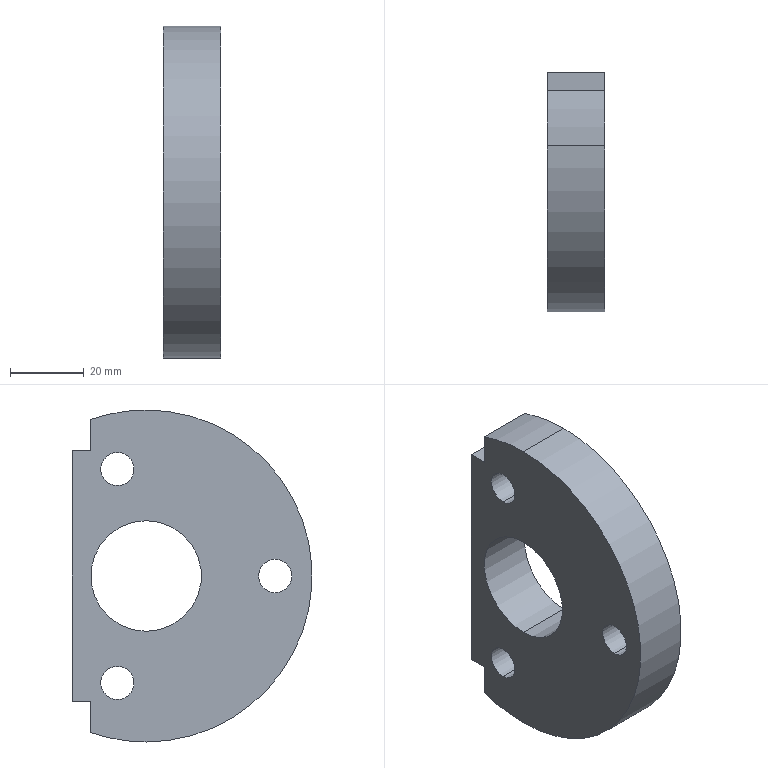Component | SolidWorks | 2SemicircularSupportPlate-1 | 1 solid | 27 faces | box 15.5 x 65 x 90 mm | volume 59022 mm3 | cylinder 17 | plane 10 | commonest cylinder face diameters 14 x6 9 x6 90 x3 30 x2
build123d program:
from build123d import *

# Parameters (mm, degrees)
BOSS_EXTRUDE1_DEPTH     = 15.5
CUT_EXTRUDE1_DEPTH      = 66.5
CUT_EXTRUDE1_DEPTH_BACK = 66.5
SKETCH2_R               = 15
HOLE1_D                 = 9
HOLE1_DEPTH             = 100
HOLE1_CBORE_D           = 14
HOLE1_CBORE_DEPTH       = 8


with BuildPart() as part:
    # Sketch1 → Boss-Extrude1 (new body)
    with BuildSketch(Plane.XY):
        with BuildLine():
            Line((-42.426, 15), (-34, 15))
            Line((-34, 15), (-34, 20))
            Line((-34, 20), (34, 20))
            Line((34, 20), (34, 15))
            Line((34, 15), (42.426, 15))
            ThreePointArc((42.426, 15), (0, -45), (-42.426, 15))
        make_face()
    extrude(amount=BOSS_EXTRUDE1_DEPTH)

    # Sketch2 → Cut-Extrude1 (cut, two sides: drawn at the far end of the back side and taken through both)
    with BuildSketch(Plane.XY.offset(15.5).offset(-CUT_EXTRUDE1_DEPTH_BACK)):
        Circle(SKETCH2_R)
    extrude(amount=CUT_EXTRUDE1_DEPTH + CUT_EXTRUDE1_DEPTH_BACK, mode=Mode.SUBTRACT)

    # Hole1
    with Locations(Plane.XY.offset(15.5)):
        with Locations((-28.978, 7.765), (28.978, 7.765), (0, -35)):
            CounterBoreHole(HOLE1_D / 2, HOLE1_CBORE_D / 2, HOLE1_CBORE_DEPTH, depth=HOLE1_DEPTH)


solid = part.part

# Placed as in the assembly
solid = solid.moved(Location((200, 65, 0), (0, 90, 0)))
STEP:
#1=COLOUR_RGB('',0.7922,0.8196,0.9333);
#2=FILL_AREA_STYLE_COLOUR('',#1);
#3=FILL_AREA_STYLE('',(#2));
#4=SURFACE_STYLE_FILL_AREA(#3);
#5=SURFACE_SIDE_STYLE('',(#4));
#6=SURFACE_STYLE_USAGE(.BOTH.,#5);
#7=PRESENTATION_STYLE_ASSIGNMENT((#6));
#8=CARTESIAN_POINT('',(8.169,1.181,0.2756));
#9=VERTEX_POINT('',#8);
#10=CARTESIAN_POINT('',(8.169,1.181,-0.2756));
#11=VERTEX_POINT('',#10);
#12=CARTESIAN_POINT('',(8.169,1.181,0.));
#13=DIRECTION('',(1.,-0.,-0.));
#14=DIRECTION('',(0.,-0.,-1.));
#15=AXIS2_PLACEMENT_3D('',#12,#13,#14);
#16=CIRCLE('',#15,0.2756);
#17=EDGE_CURVE('',#9,#11,#16,.T.);
#18=ORIENTED_EDGE('',*,*,#17,.F.);
#19=CARTESIAN_POINT('',(8.484,1.181,0.2756));
#20=VERTEX_POINT('',#19);
#21=CARTESIAN_POINT('',(8.484,1.181,0.2756));
#22=DIRECTION('',(1.,-0.,-0.));
#23=VECTOR('',#22,39.37);
#24=LINE('',#21,#23);
#25=EDGE_CURVE('',#9,#20,#24,.T.);
#26=ORIENTED_EDGE('',*,*,#25,.T.);
#27=CARTESIAN_POINT('',(8.484,1.181,-0.2756));
#28=VERTEX_POINT('',#27);
#29=CARTESIAN_POINT('',(8.484,1.181,0.));
#30=DIRECTION('',(1.,-0.,-0.));
#31=DIRECTION('',(0.,-0.,-1.));
#32=AXIS2_PLACEMENT_3D('',#29,#30,#31);
#33=CIRCLE('',#32,0.2756);
#34=EDGE_CURVE('',#20,#28,#33,.T.);
#35=ORIENTED_EDGE('',*,*,#34,.T.);
#36=CARTESIAN_POINT('',(8.484,1.181,-0.2756));
#37=DIRECTION('',(1.,-0.,-0.));
#38=VECTOR('',#37,39.37);
#39=LINE('',#36,#38);
#40=EDGE_CURVE('',#11,#28,#39,.T.);
#41=ORIENTED_EDGE('',*,*,#40,.F.);
#42=EDGE_LOOP('',(#18,#26,#35,#41));
#43=FACE_OUTER_BOUND('',#42,.T.);
#44=CARTESIAN_POINT('',(8.484,1.181,0.));
#45=DIRECTION('',(1.,-0.,-0.));
#46=DIRECTION('',(0.,-0.,-1.));
#47=AXIS2_PLACEMENT_3D('',#44,#45,#46);
#48=CYLINDRICAL_SURFACE('',#47,0.2756);
#49=ADVANCED_FACE('',(#43),#48,.F.);
#50=CARTESIAN_POINT('',(7.874,1.181,0.1772));
#51=VERTEX_POINT('',#50);
#52=CARTESIAN_POINT('',(7.874,1.181,-0.1772));
#53=VERTEX_POINT('',#52);
#54=CARTESIAN_POINT('',(7.874,1.181,0.));
#55=DIRECTION('',(1.,-0.,-0.));
#56=DIRECTION('',(0.,-0.,-1.));
#57=AXIS2_PLACEMENT_3D('',#54,#55,#56);
#58=CIRCLE('',#57,0.1772);
#59=EDGE_CURVE('',#51,#53,#58,.T.);
#60=ORIENTED_EDGE('',*,*,#59,.F.);
#61=CARTESIAN_POINT('',(8.169,1.181,0.1772));
#62=VERTEX_POINT('',#61);
#63=CARTESIAN_POINT('',(8.484,1.181,0.1772));
#64=DIRECTION('',(1.,-0.,-0.));
#65=VECTOR('',#64,39.37);
#66=LINE('',#63,#65);
#67=EDGE_CURVE('',#51,#62,#66,.T.);
#68=ORIENTED_EDGE('',*,*,#67,.T.);
#69=CARTESIAN_POINT('',(8.169,1.181,-0.1772));
#70=VERTEX_POINT('',#69);
#71=CARTESIAN_POINT('',(8.169,1.181,0.));
#72=DIRECTION('',(1.,-0.,-0.));
#73=DIRECTION('',(0.,-0.,-1.));
#74=AXIS2_PLACEMENT_3D('',#71,#72,#73);
#75=CIRCLE('',#74,0.1772);
#76=EDGE_CURVE('',#62,#70,#75,.T.);
#77=ORIENTED_EDGE('',*,*,#76,.T.);
#78=CARTESIAN_POINT('',(8.484,1.181,-0.1772));
#79=DIRECTION('',(1.,-0.,-0.));
#80=VECTOR('',#79,39.37);
#81=LINE('',#78,#80);
#82=EDGE_CURVE('',#53,#70,#81,.T.);
#83=ORIENTED_EDGE('',*,*,#82,.F.);
#84=EDGE_LOOP('',(#60,#68,#77,#83));
#85=FACE_OUTER_BOUND('',#84,.T.);
#86=CARTESIAN_POINT('',(8.484,1.181,0.));
#87=DIRECTION('',(1.,-0.,-0.));
#88=DIRECTION('',(0.,-0.,-1.));
#89=AXIS2_PLACEMENT_3D('',#86,#87,#88);
#90=CYLINDRICAL_SURFACE('',#89,0.1772);
#91=ADVANCED_FACE('',(#85),#90,.F.);
#92=CARTESIAN_POINT('',(8.169,2.865,-0.8653));
#93=VERTEX_POINT('',#92);
#94=CARTESIAN_POINT('',(8.169,2.865,-1.416));
#95=VERTEX_POINT('',#94);
#96=CARTESIAN_POINT('',(8.169,2.865,-1.141));
#97=DIRECTION('',(1.,-0.,-0.));
#98=DIRECTION('',(0.,-0.,-1.));
#99=AXIS2_PLACEMENT_3D('',#96,#97,#98);
#100=CIRCLE('',#99,0.2756);
#101=EDGE_CURVE('',#93,#95,#100,.T.);
#102=ORIENTED_EDGE('',*,*,#101,.F.);
#103=CARTESIAN_POINT('',(8.484,2.865,-0.8653));
#104=VERTEX_POINT('',#103);
#105=CARTESIAN_POINT('',(8.484,2.865,-0.8653));
#106=DIRECTION('',(1.,-0.,-0.));
#107=VECTOR('',#106,39.37);
#108=LINE('',#105,#107);
#109=EDGE_CURVE('',#93,#104,#108,.T.);
#110=ORIENTED_EDGE('',*,*,#109,.T.);
#111=CARTESIAN_POINT('',(8.484,2.865,-1.416));
#112=VERTEX_POINT('',#111);
#113=CARTESIAN_POINT('',(8.484,2.865,-1.141));
#114=DIRECTION('',(1.,-0.,-0.));
#115=DIRECTION('',(0.,-0.,-1.));
#116=AXIS2_PLACEMENT_3D('',#113,#114,#115);
#117=CIRCLE('',#116,0.2756);
#118=EDGE_CURVE('',#104,#112,#117,.T.);
#119=ORIENTED_EDGE('',*,*,#118,.T.);
#120=CARTESIAN_POINT('',(8.484,2.865,-1.416));
#121=DIRECTION('',(1.,-0.,-0.));
#122=VECTOR('',#121,39.37);
#123=LINE('',#120,#122);
#124=EDGE_CURVE('',#95,#112,#123,.T.);
#125=ORIENTED_EDGE('',*,*,#124,.F.);
#126=EDGE_LOOP('',(#102,#110,#119,#125));
#127=FACE_OUTER_BOUND('',#126,.T.);
#128=CARTESIAN_POINT('',(8.484,2.865,-1.141));
#129=DIRECTION('',(1.,-0.,-0.));
#130=DIRECTION('',(0.,-0.,-1.));
#131=AXIS2_PLACEMENT_3D('',#128,#129,#130);
#132=CYLINDRICAL_SURFACE('',#131,0.2756);
#133=ADVANCED_FACE('',(#127),#132,.F.);
#134=CARTESIAN_POINT('',(7.874,2.865,-0.9637));
#135=VERTEX_POINT('',#134);
#136=CARTESIAN_POINT('',(7.874,2.865,-1.318));
#137=VERTEX_POINT('',#136);
#138=CARTESIAN_POINT('',(7.874,2.865,-1.141));
#139=DIRECTION('',(1.,-0.,-0.));
#140=DIRECTION('',(0.,-0.,-1.));
#141=AXIS2_PLACEMENT_3D('',#138,#139,#140);
#142=CIRCLE('',#141,0.1772);
#143=EDGE_CURVE('',#135,#137,#142,.T.);
#144=ORIENTED_EDGE('',*,*,#143,.F.);
#145=CARTESIAN_POINT('',(8.169,2.865,-0.9637));
#146=VERTEX_POINT('',#145);
#147=CARTESIAN_POINT('',(8.484,2.865,-0.9637));
#148=DIRECTION('',(1.,-0.,-0.));
#149=VECTOR('',#148,39.37);
#150=LINE('',#147,#149);
#151=EDGE_CURVE('',#135,#146,#150,.T.);
#152=ORIENTED_EDGE('',*,*,#151,.T.);
#153=CARTESIAN_POINT('',(8.169,2.865,-1.318));
#154=VERTEX_POINT('',#153);
#155=CARTESIAN_POINT('',(8.169,2.865,-1.141));
#156=DIRECTION('',(1.,-0.,-0.));
#157=DIRECTION('',(0.,-0.,-1.));
#158=AXIS2_PLACEMENT_3D('',#155,#156,#157);
#159=CIRCLE('',#158,0.1772);
#160=EDGE_CURVE('',#146,#154,#159,.T.);
#161=ORIENTED_EDGE('',*,*,#160,.T.);
#162=CARTESIAN_POINT('',(8.484,2.865,-1.318));
#163=DIRECTION('',(1.,-0.,-0.));
#164=VECTOR('',#163,39.37);
#165=LINE('',#162,#164);
#166=EDGE_CURVE('',#137,#154,#165,.T.);
#167=ORIENTED_EDGE('',*,*,#166,.F.);
#168=EDGE_LOOP('',(#144,#152,#161,#167));
#169=FACE_OUTER_BOUND('',#168,.T.);
#170=CARTESIAN_POINT('',(8.484,2.865,-1.141));
#171=DIRECTION('',(1.,-0.,-0.));
#172=DIRECTION('',(0.,-0.,-1.));
#173=AXIS2_PLACEMENT_3D('',#170,#171,#172);
#174=CYLINDRICAL_SURFACE('',#173,0.1772);
#175=ADVANCED_FACE('',(#169),#174,.F.);
#176=CARTESIAN_POINT('',(8.169,2.865,1.416));
#177=VERTEX_POINT('',#176);
#178=CARTESIAN_POINT('',(8.169,2.865,0.8653));
#179=VERTEX_POINT('',#178);
#180=CARTESIAN_POINT('',(8.169,2.865,1.141));
#181=DIRECTION('',(1.,-0.,-0.));
#182=DIRECTION('',(0.,-0.,-1.));
#183=AXIS2_PLACEMENT_3D('',#180,#181,#182);
#184=CIRCLE('',#183,0.2756);
#185=EDGE_CURVE('',#177,#179,#184,.T.);
#186=ORIENTED_EDGE('',*,*,#185,.F.);
#187=CARTESIAN_POINT('',(8.484,2.865,1.416));
#188=VERTEX_POINT('',#187);
#189=CARTESIAN_POINT('',(8.484,2.865,1.416));
#190=DIRECTION('',(1.,-0.,-0.));
#191=VECTOR('',#190,39.37);
#192=LINE('',#189,#191);
#193=EDGE_CURVE('',#177,#188,#192,.T.);
#194=ORIENTED_EDGE('',*,*,#193,.T.);
#195=CARTESIAN_POINT('',(8.484,2.865,0.8653));
#196=VERTEX_POINT('',#195);
#197=CARTESIAN_POINT('',(8.484,2.865,1.141));
#198=DIRECTION('',(1.,-0.,-0.));
#199=DIRECTION('',(0.,-0.,-1.));
#200=AXIS2_PLACEMENT_3D('',#197,#198,#199);
#201=CIRCLE('',#200,0.2756);
#202=EDGE_CURVE('',#188,#196,#201,.T.);
#203=ORIENTED_EDGE('',*,*,#202,.T.);
#204=CARTESIAN_POINT('',(8.484,2.865,0.8653));
#205=DIRECTION('',(1.,-0.,-0.));
#206=VECTOR('',#205,39.37);
#207=LINE('',#204,#206);
#208=EDGE_CURVE('',#179,#196,#207,.T.);
#209=ORIENTED_EDGE('',*,*,#208,.F.);
#210=EDGE_LOOP('',(#186,#194,#203,#209));
#211=FACE_OUTER_BOUND('',#210,.T.);
#212=CARTESIAN_POINT('',(8.484,2.865,1.141));
#213=DIRECTION('',(1.,-0.,-0.));
#214=DIRECTION('',(0.,-0.,-1.));
#215=AXIS2_PLACEMENT_3D('',#212,#213,#214);
#216=CYLINDRICAL_SURFACE('',#215,0.2756);
#217=ADVANCED_FACE('',(#211),#216,.F.);
#218=CARTESIAN_POINT('',(7.874,2.865,1.318));
#219=VERTEX_POINT('',#218);
#220=CARTESIAN_POINT('',(7.874,2.865,0.9637));
#221=VERTEX_POINT('',#220);
#222=CARTESIAN_POINT('',(7.874,2.865,1.141));
#223=DIRECTION('',(1.,-0.,-0.));
#224=DIRECTION('',(0.,-0.,-1.));
#225=AXIS2_PLACEMENT_3D('',#222,#223,#224);
#226=CIRCLE('',#225,0.1772);
#227=EDGE_CURVE('',#219,#221,#226,.T.);
#228=ORIENTED_EDGE('',*,*,#227,.F.);
#229=CARTESIAN_POINT('',(8.169,2.865,1.318));
#230=VERTEX_POINT('',#229);
#231=CARTESIAN_POINT('',(8.484,2.865,1.318));
#232=DIRECTION('',(1.,-0.,-0.));
#233=VECTOR('',#232,39.37);
#234=LINE('',#231,#233);
#235=EDGE_CURVE('',#219,#230,#234,.T.);
#236=ORIENTED_EDGE('',*,*,#235,.T.);
#237=CARTESIAN_POINT('',(8.169,2.865,0.9637));
#238=VERTEX_POINT('',#237);
#239=CARTESIAN_POINT('',(8.169,2.865,1.141));
#240=DIRECTION('',(1.,-0.,-0.));
#241=DIRECTION('',(0.,-0.,-1.));
#242=AXIS2_PLACEMENT_3D('',#239,#240,#241);
#243=CIRCLE('',#242,0.1772);
#244=EDGE_CURVE('',#230,#238,#243,.T.);
#245=ORIENTED_EDGE('',*,*,#244,.T.);
#246=CARTESIAN_POINT('',(8.484,2.865,0.9637));
#247=DIRECTION('',(1.,-0.,-0.));
#248=VECTOR('',#247,39.37);
#249=LINE('',#246,#248);
#250=EDGE_CURVE('',#221,#238,#249,.T.);
#251=ORIENTED_EDGE('',*,*,#250,.F.);
#252=EDGE_LOOP('',(#228,#236,#245,#251));
#253=FACE_OUTER_BOUND('',#252,.T.);
#254=CARTESIAN_POINT('',(8.484,2.865,1.141));
#255=DIRECTION('',(1.,-0.,-0.));
#256=DIRECTION('',(0.,-0.,-1.));
#257=AXIS2_PLACEMENT_3D('',#254,#255,#256);
#258=CYLINDRICAL_SURFACE('',#257,0.1772);
#259=ADVANCED_FACE('',(#253),#258,.F.);
#260=CARTESIAN_POINT('',(7.874,2.559,0.5906));
#261=VERTEX_POINT('',#260);
#262=CARTESIAN_POINT('',(7.874,2.559,-0.5906));
#263=VERTEX_POINT('',#262);
#264=CARTESIAN_POINT('',(7.874,2.559,-0.));
#265=DIRECTION('',(1.,-0.,-0.));
#266=DIRECTION('',(0.,-0.,-1.));
#267=AXIS2_PLACEMENT_3D('',#264,#265,#266);
#268=CIRCLE('',#267,0.5906);
#269=EDGE_CURVE('',#261,#263,#268,.T.);
#270=ORIENTED_EDGE('',*,*,#269,.F.);
#271=CARTESIAN_POINT('',(8.484,2.559,0.5906));
#272=VERTEX_POINT('',#271);
#273=CARTESIAN_POINT('',(7.874,2.559,0.5906));
#274=DIRECTION('',(1.,-0.,-0.));
#275=VECTOR('',#274,39.37);
#276=LINE('',#273,#275);
#277=EDGE_CURVE('',#261,#272,#276,.T.);
#278=ORIENTED_EDGE('',*,*,#277,.T.);
#279=CARTESIAN_POINT('',(8.484,2.559,-0.5906));
#280=VERTEX_POINT('',#279);
#281=CARTESIAN_POINT('',(8.484,2.559,-0.));
#282=DIRECTION('',(1.,-0.,-0.));
#283=DIRECTION('',(0.,-0.,-1.));
#284=AXIS2_PLACEMENT_3D('',#281,#282,#283);
#285=CIRCLE('',#284,0.5906);
#286=EDGE_CURVE('',#272,#280,#285,.T.);
#287=ORIENTED_EDGE('',*,*,#286,.T.);
#288=CARTESIAN_POINT('',(7.874,2.559,-0.5906));
#289=DIRECTION('',(1.,-0.,-0.));
#290=VECTOR('',#289,39.37);
#291=LINE('',#288,#290);
#292=EDGE_CURVE('',#263,#280,#291,.T.);
#293=ORIENTED_EDGE('',*,*,#292,.F.);
#294=EDGE_LOOP('',(#270,#278,#287,#293));
#295=FACE_OUTER_BOUND('',#294,.T.);
#296=CARTESIAN_POINT('',(7.874,2.559,-0.));
#297=DIRECTION('',(1.,-0.,-0.));
#298=DIRECTION('',(0.,-0.,-1.));
#299=AXIS2_PLACEMENT_3D('',#296,#297,#298);
#300=CYLINDRICAL_SURFACE('',#299,0.5906);
#301=ADVANCED_FACE('',(#295),#300,.F.);
#302=CARTESIAN_POINT('',(8.484,2.559,-1.772));
#303=VERTEX_POINT('',#302);
#304=CARTESIAN_POINT('',(8.484,3.15,-1.67));
#305=VERTEX_POINT('',#304);
#306=CARTESIAN_POINT('',(8.484,2.559,-0.));
#307=DIRECTION('',(1.,-0.,-0.));
#308=DIRECTION('',(-0.,-0.,-1.));
#309=AXIS2_PLACEMENT_3D('',#306,#307,#308);
#310=CIRCLE('',#309,1.772);
#311=EDGE_CURVE('',#303,#305,#310,.T.);
#312=ORIENTED_EDGE('',*,*,#311,.F.);
#313=CARTESIAN_POINT('',(7.874,2.559,-1.772));
#314=VERTEX_POINT('',#313);
#315=CARTESIAN_POINT('',(8.484,2.559,-1.772));
#316=DIRECTION('',(-1.,0.,0.));
#317=VECTOR('',#316,39.37);
#318=LINE('',#315,#317);
#319=EDGE_CURVE('',#303,#314,#318,.T.);
#320=ORIENTED_EDGE('',*,*,#319,.T.);
#321=CARTESIAN_POINT('',(7.874,3.15,-1.67));
#322=VERTEX_POINT('',#321);
#323=CARTESIAN_POINT('',(7.874,2.559,-0.));
#324=DIRECTION('',(1.,-0.,-0.));
#325=DIRECTION('',(-0.,-0.,-1.));
#326=AXIS2_PLACEMENT_3D('',#323,#324,#325);
#327=CIRCLE('',#326,1.772);
#328=EDGE_CURVE('',#314,#322,#327,.T.);
#329=ORIENTED_EDGE('',*,*,#328,.T.);
#330=CARTESIAN_POINT('',(8.484,3.15,-1.67));
#331=DIRECTION('',(-1.,0.,0.));
#332=VECTOR('',#331,39.37);
#333=LINE('',#330,#332);
#334=EDGE_CURVE('',#305,#322,#333,.T.);
#335=ORIENTED_EDGE('',*,*,#334,.F.);
#336=EDGE_LOOP('',(#312,#320,#329,#335));
#337=FACE_OUTER_BOUND('',#336,.T.);
#338=CARTESIAN_POINT('',(8.484,2.559,-0.));
#339=DIRECTION('',(-1.,0.,0.));
#340=DIRECTION('',(0.,0.,1.));
#341=AXIS2_PLACEMENT_3D('',#338,#339,#340);
#342=CYLINDRICAL_SURFACE('',#341,1.772);
#343=ADVANCED_FACE('',(#337),#342,.T.);
#344=ORIENTED_EDGE('',*,*,#319,.F.);
#345=CARTESIAN_POINT('',(8.484,2.559,1.772));
#346=VERTEX_POINT('',#345);
#347=CARTESIAN_POINT('',(8.484,2.559,-0.));
#348=DIRECTION('',(1.,-0.,-0.));
#349=DIRECTION('',(-0.,-0.,-1.));
#350=AXIS2_PLACEMENT_3D('',#347,#348,#349);
#351=CIRCLE('',#350,1.772);
#352=EDGE_CURVE('',#346,#303,#351,.T.);
#353=ORIENTED_EDGE('',*,*,#352,.F.);
#354=CARTESIAN_POINT('',(7.874,2.559,1.772));
#355=VERTEX_POINT('',#354);
#356=CARTESIAN_POINT('',(8.484,2.559,1.772));
#357=DIRECTION('',(-1.,0.,0.));
#358=VECTOR('',#357,39.37);
#359=LINE('',#356,#358);
#360=EDGE_CURVE('',#346,#355,#359,.T.);
#361=ORIENTED_EDGE('',*,*,#360,.T.);
#362=CARTESIAN_POINT('',(7.874,2.559,-0.));
#363=DIRECTION('',(1.,-0.,-0.));
#364=DIRECTION('',(-0.,-0.,-1.));
#365=AXIS2_PLACEMENT_3D('',#362,#363,#364);
#366=CIRCLE('',#365,1.772);
#367=EDGE_CURVE('',#355,#314,#366,.T.);
#368=ORIENTED_EDGE('',*,*,#367,.T.);
#369=EDGE_LOOP('',(#344,#353,#361,#368));
#370=FACE_OUTER_BOUND('',#369,.T.);
#371=CARTESIAN_POINT('',(8.484,2.559,-0.));
#372=DIRECTION('',(-1.,0.,0.));
#373=DIRECTION('',(0.,0.,1.));
#374=AXIS2_PLACEMENT_3D('',#371,#372,#373);
#375=CYLINDRICAL_SURFACE('',#374,1.772);
#376=ADVANCED_FACE('',(#370),#375,.T.);
#377=ORIENTED_EDGE('',*,*,#360,.F.);
#378=CARTESIAN_POINT('',(8.484,3.15,1.67));
#379=VERTEX_POINT('',#378);
#380=CARTESIAN_POINT('',(8.484,2.559,-0.));
#381=DIRECTION('',(1.,-0.,-0.));
#382=DIRECTION('',(-0.,-0.,-1.));
#383=AXIS2_PLACEMENT_3D('',#380,#381,#382);
#384=CIRCLE('',#383,1.772);
#385=EDGE_CURVE('',#379,#346,#384,.T.);
#386=ORIENTED_EDGE('',*,*,#385,.F.);
#387=CARTESIAN_POINT('',(7.874,3.15,1.67));
#388=VERTEX_POINT('',#387);
#389=CARTESIAN_POINT('',(8.484,3.15,1.67));
#390=DIRECTION('',(-1.,0.,0.));
#391=VECTOR('',#390,39.37);
#392=LINE('',#389,#391);
#393=EDGE_CURVE('',#379,#388,#392,.T.);
#394=ORIENTED_EDGE('',*,*,#393,.T.);
#395=CARTESIAN_POINT('',(7.874,2.559,-0.));
#396=DIRECTION('',(1.,-0.,-0.));
#397=DIRECTION('',(-0.,-0.,-1.));
#398=AXIS2_PLACEMENT_3D('',#395,#396,#397);
#399=CIRCLE('',#398,1.772);
#400=EDGE_CURVE('',#388,#355,#399,.T.);
#401=ORIENTED_EDGE('',*,*,#400,.T.);
#402=EDGE_LOOP('',(#377,#386,#394,#401));
#403=FACE_OUTER_BOUND('',#402,.T.);
#404=CARTESIAN_POINT('',(8.484,2.559,-0.));
#405=DIRECTION('',(-1.,0.,0.));
#406=DIRECTION('',(0.,0.,1.));
#407=AXIS2_PLACEMENT_3D('',#404,#405,#406);
#408=CYLINDRICAL_SURFACE('',#407,1.772);
#409=ADVANCED_FACE('',(#403),#408,.T.);
#410=CARTESIAN_POINT('',(7.874,3.15,-1.339));
#411=VERTEX_POINT('',#410);
#412=CARTESIAN_POINT('',(7.874,3.15,-1.67));
#413=DIRECTION('',(0.,0.,1.));
#414=VECTOR('',#413,39.37);
#415=LINE('',#412,#414);
#416=EDGE_CURVE('',#322,#411,#415,.T.);
#417=ORIENTED_EDGE('',*,*,#416,.T.);
#418=CARTESIAN_POINT('',(8.484,3.15,-1.339));
#419=VERTEX_POINT('',#418);
#420=CARTESIAN_POINT('',(8.484,3.15,-1.339));
#421=DIRECTION('',(-1.,0.,0.));
#422=VECTOR('',#421,39.37);
#423=LINE('',#420,#422);
#424=EDGE_CURVE('',#419,#411,#423,.T.);
#425=ORIENTED_EDGE('',*,*,#424,.F.);
#426=CARTESIAN_POINT('',(8.484,3.15,-1.67));
#427=DIRECTION('',(0.,0.,1.));
#428=VECTOR('',#427,39.37);
#429=LINE('',#426,#428);
#430=EDGE_CURVE('',#305,#419,#429,.T.);
#431=ORIENTED_EDGE('',*,*,#430,.F.);
#432=ORIENTED_EDGE('',*,*,#334,.T.);
#433=EDGE_LOOP('',(#417,#425,#431,#432));
#434=FACE_OUTER_BOUND('',#433,.T.);
#435=CARTESIAN_POINT('',(8.484,3.15,-1.67));
#436=DIRECTION('',(-0.,-1.,0.));
#437=DIRECTION('',(-0.,-0.,-1.));
#438=AXIS2_PLACEMENT_3D('',#435,#436,#437);
#439=PLANE('',#438);
#440=ADVANCED_FACE('',(#434),#439,.F.);
#441=CARTESIAN_POINT('',(7.874,3.346,-1.339));
#442=VERTEX_POINT('',#441);
#443=CARTESIAN_POINT('',(7.874,3.15,-1.339));
#444=DIRECTION('',(0.,1.,-0.));
#445=VECTOR('',#444,39.37);
#446=LINE('',#443,#445);
#447=EDGE_CURVE('',#411,#442,#446,.T.);
#448=ORIENTED_EDGE('',*,*,#447,.T.);
#449=CARTESIAN_POINT('',(8.484,3.346,-1.339));
#450=VERTEX_POINT('',#449);
#451=CARTESIAN_POINT('',(8.484,3.346,-1.339));
#452=DIRECTION('',(-1.,0.,0.));
#453=VECTOR('',#452,39.37);
#454=LINE('',#451,#453);
#455=EDGE_CURVE('',#450,#442,#454,.T.);
#456=ORIENTED_EDGE('',*,*,#455,.F.);
#457=CARTESIAN_POINT('',(8.484,3.15,-1.339));
#458=DIRECTION('',(0.,1.,-0.));
#459=VECTOR('',#458,39.37);
#460=LINE('',#457,#459);
#461=EDGE_CURVE('',#419,#450,#460,.T.);
#462=ORIENTED_EDGE('',*,*,#461,.F.);
#463=ORIENTED_EDGE('',*,*,#424,.T.);
#464=EDGE_LOOP('',(#448,#456,#462,#463));
#465=FACE_OUTER_BOUND('',#464,.T.);
#466=CARTESIAN_POINT('',(8.484,3.15,-1.339));
#467=DIRECTION('',(0.,0.,1.));
#468=DIRECTION('',(1.,-0.,-0.));
#469=AXIS2_PLACEMENT_3D('',#466,#467,#468);
#470=PLANE('',#469);
#471=ADVANCED_FACE('',(#465),#470,.F.);
#472=CARTESIAN_POINT('',(7.874,3.346,1.339));
#473=VERTEX_POINT('',#472);
#474=CARTESIAN_POINT('',(7.874,3.346,1.339));
#475=DIRECTION('',(0.,0.,1.));
#476=VECTOR('',#475,39.37);
#477=LINE('',#474,#476);
#478=EDGE_CURVE('',#442,#473,#477,.T.);
#479=ORIENTED_EDGE('',*,*,#478,.T.);
#480=CARTESIAN_POINT('',(8.484,3.346,1.339));
#481=VERTEX_POINT('',#480);
#482=CARTESIAN_POINT('',(8.484,3.346,1.339));
#483=DIRECTION('',(-1.,0.,0.));
#484=VECTOR('',#483,39.37);
#485=LINE('',#482,#484);
#486=EDGE_CURVE('',#481,#473,#485,.T.);
#487=ORIENTED_EDGE('',*,*,#486,.F.);
#488=CARTESIAN_POINT('',(8.484,3.346,1.339));
#489=DIRECTION('',(0.,0.,1.));
#490=VECTOR('',#489,39.37);
#491=LINE('',#488,#490);
#492=EDGE_CURVE('',#450,#481,#491,.T.);
#493=ORIENTED_EDGE('',*,*,#492,.F.);
#494=ORIENTED_EDGE('',*,*,#455,.T.);
#495=EDGE_LOOP('',(#479,#487,#493,#494));
#496=FACE_OUTER_BOUND('',#495,.T.);
#497=CARTESIAN_POINT('',(8.484,3.346,1.339));
#498=DIRECTION('',(-0.,-1.,0.));
#499=DIRECTION('',(-0.,-0.,-1.));
#500=AXIS2_PLACEMENT_3D('',#497,#498,#499);
#501=PLANE('',#500);
#502=ADVANCED_FACE('',(#496),#501,.F.);
#503=CARTESIAN_POINT('',(7.874,3.15,1.339));
#504=VERTEX_POINT('',#503);
#505=CARTESIAN_POINT('',(7.874,3.15,1.339));
#506=DIRECTION('',(-0.,-1.,0.));
#507=VECTOR('',#506,39.37);
#508=LINE('',#505,#507);
#509=EDGE_CURVE('',#473,#504,#508,.T.);
#510=ORIENTED_EDGE('',*,*,#509,.T.);
#511=CARTESIAN_POINT('',(8.484,3.15,1.339));
#512=VERTEX_POINT('',#511);
#513=CARTESIAN_POINT('',(8.484,3.15,1.339));
#514=DIRECTION('',(-1.,0.,0.));
#515=VECTOR('',#514,39.37);
#516=LINE('',#513,#515);
#517=EDGE_CURVE('',#512,#504,#516,.T.);
#518=ORIENTED_EDGE('',*,*,#517,.F.);
#519=CARTESIAN_POINT('',(8.484,3.15,1.339));
#520=DIRECTION('',(-0.,-1.,0.));
#521=VECTOR('',#520,39.37);
#522=LINE('',#519,#521);
#523=EDGE_CURVE('',#481,#512,#522,.T.);
#524=ORIENTED_EDGE('',*,*,#523,.F.);
#525=ORIENTED_EDGE('',*,*,#486,.T.);
#526=EDGE_LOOP('',(#510,#518,#524,#525));
#527=FACE_OUTER_BOUND('',#526,.T.);
#528=CARTESIAN_POINT('',(8.484,3.15,1.339));
#529=DIRECTION('',(-0.,-0.,-1.));
#530=DIRECTION('',(-1.,0.,0.));
#531=AXIS2_PLACEMENT_3D('',#528,#529,#530);
#532=PLANE('',#531);
#533=ADVANCED_FACE('',(#527),#532,.F.);
#534=CARTESIAN_POINT('',(7.874,3.15,1.67));
#535=DIRECTION('',(0.,0.,1.));
#536=VECTOR('',#535,39.37);
#537=LINE('',#534,#536);
#538=EDGE_CURVE('',#504,#388,#537,.T.);
#539=ORIENTED_EDGE('',*,*,#538,.T.);
#540=ORIENTED_EDGE('',*,*,#393,.F.);
#541=CARTESIAN_POINT('',(8.484,3.15,1.67));
#542=DIRECTION('',(0.,0.,1.));
#543=VECTOR('',#542,39.37);
#544=LINE('',#541,#543);
#545=EDGE_CURVE('',#512,#379,#544,.T.);
#546=ORIENTED_EDGE('',*,*,#545,.F.);
#547=ORIENTED_EDGE('',*,*,#517,.T.);
#548=EDGE_LOOP('',(#539,#540,#546,#547));
#549=FACE_OUTER_BOUND('',#548,.T.);
#550=CARTESIAN_POINT('',(8.484,3.15,1.67));
#551=DIRECTION('',(-0.,-1.,0.));
#552=DIRECTION('',(-0.,-0.,-1.));
#553=AXIS2_PLACEMENT_3D('',#550,#551,#552);
#554=PLANE('',#553);
#555=ADVANCED_FACE('',(#549),#554,.F.);
#556=CARTESIAN_POINT('',(8.484,1.181,0.));
#557=DIRECTION('',(1.,-0.,-0.));
#558=DIRECTION('',(0.,-0.,-1.));
#559=AXIS2_PLACEMENT_3D('',#556,#557,#558);
#560=CIRCLE('',#559,0.2756);
#561=EDGE_CURVE('',#28,#20,#560,.T.);
#562=ORIENTED_EDGE('',*,*,#561,.F.);
#563=ORIENTED_EDGE('',*,*,#34,.F.);
#564=EDGE_LOOP('',(#562,#563));
#565=FACE_BOUND('',#564,.T.);
#566=CARTESIAN_POINT('',(8.484,2.865,-1.141));
#567=DIRECTION('',(1.,-0.,-0.));
#568=DIRECTION('',(0.,-0.,-1.));
#569=AXIS2_PLACEMENT_3D('',#566,#567,#568);
#570=CIRCLE('',#569,0.2756);
#571=EDGE_CURVE('',#112,#104,#570,.T.);
#572=ORIENTED_EDGE('',*,*,#571,.F.);
#573=ORIENTED_EDGE('',*,*,#118,.F.);
#574=EDGE_LOOP('',(#572,#573));
#575=FACE_BOUND('',#574,.T.);
#576=CARTESIAN_POINT('',(8.484,2.865,1.141));
#577=DIRECTION('',(1.,-0.,-0.));
#578=DIRECTION('',(0.,-0.,-1.));
#579=AXIS2_PLACEMENT_3D('',#576,#577,#578);
#580=CIRCLE('',#579,0.2756);
#581=EDGE_CURVE('',#196,#188,#580,.T.);
#582=ORIENTED_EDGE('',*,*,#581,.F.);
#583=ORIENTED_EDGE('',*,*,#202,.F.);
#584=EDGE_LOOP('',(#582,#583));
#585=FACE_BOUND('',#584,.T.);
#586=CARTESIAN_POINT('',(8.484,2.559,-0.));
#587=DIRECTION('',(1.,-0.,-0.));
#588=DIRECTION('',(0.,-0.,-1.));
#589=AXIS2_PLACEMENT_3D('',#586,#587,#588);
#590=CIRCLE('',#589,0.5906);
#591=EDGE_CURVE('',#280,#272,#590,.T.);
#592=ORIENTED_EDGE('',*,*,#591,.F.);
#593=ORIENTED_EDGE('',*,*,#286,.F.);
#594=EDGE_LOOP('',(#592,#593));
#595=FACE_BOUND('',#594,.T.);
#596=ORIENTED_EDGE('',*,*,#385,.T.);
#597=ORIENTED_EDGE('',*,*,#352,.T.);
#598=ORIENTED_EDGE('',*,*,#311,.T.);
#599=ORIENTED_EDGE('',*,*,#430,.T.);
#600=ORIENTED_EDGE('',*,*,#461,.T.);
#601=ORIENTED_EDGE('',*,*,#492,.T.);
#602=ORIENTED_EDGE('',*,*,#523,.T.);
#603=ORIENTED_EDGE('',*,*,#545,.T.);
#604=EDGE_LOOP('',(#596,#597,#598,#599,#600,#601,#602,#603));
#605=FACE_OUTER_BOUND('',#604,.T.);
#606=CARTESIAN_POINT('',(8.484,2.559,-0.));
#607=DIRECTION('',(1.,-0.,-0.));
#608=DIRECTION('',(-0.,-0.,-1.));
#609=AXIS2_PLACEMENT_3D('',#606,#607,#608);
#610=PLANE('',#609);
#611=ADVANCED_FACE('',(#565,#575,#585,#595,#605),#610,.T.);
#612=CARTESIAN_POINT('',(7.874,1.181,0.));
#613=DIRECTION('',(1.,-0.,-0.));
#614=DIRECTION('',(0.,-0.,-1.));
#615=AXIS2_PLACEMENT_3D('',#612,#613,#614);
#616=CIRCLE('',#615,0.1772);
#617=EDGE_CURVE('',#53,#51,#616,.T.);
#618=ORIENTED_EDGE('',*,*,#617,.T.);
#619=ORIENTED_EDGE('',*,*,#59,.T.);
#620=EDGE_LOOP('',(#618,#619));
#621=FACE_BOUND('',#620,.T.);
#622=CARTESIAN_POINT('',(7.874,2.865,-1.141));
#623=DIRECTION('',(1.,-0.,-0.));
#624=DIRECTION('',(0.,-0.,-1.));
#625=AXIS2_PLACEMENT_3D('',#622,#623,#624);
#626=CIRCLE('',#625,0.1772);
#627=EDGE_CURVE('',#137,#135,#626,.T.);
#628=ORIENTED_EDGE('',*,*,#627,.T.);
#629=ORIENTED_EDGE('',*,*,#143,.T.);
#630=EDGE_LOOP('',(#628,#629));
#631=FACE_BOUND('',#630,.T.);
#632=CARTESIAN_POINT('',(7.874,2.865,1.141));
#633=DIRECTION('',(1.,-0.,-0.));
#634=DIRECTION('',(0.,-0.,-1.));
#635=AXIS2_PLACEMENT_3D('',#632,#633,#634);
#636=CIRCLE('',#635,0.1772);
#637=EDGE_CURVE('',#221,#219,#636,.T.);
#638=ORIENTED_EDGE('',*,*,#637,.T.);
#639=ORIENTED_EDGE('',*,*,#227,.T.);
#640=EDGE_LOOP('',(#638,#639));
#641=FACE_BOUND('',#640,.T.);
#642=CARTESIAN_POINT('',(7.874,2.559,-0.));
#643=DIRECTION('',(1.,-0.,-0.));
#644=DIRECTION('',(0.,-0.,-1.));
#645=AXIS2_PLACEMENT_3D('',#642,#643,#644);
#646=CIRCLE('',#645,0.5906);
#647=EDGE_CURVE('',#263,#261,#646,.T.);
#648=ORIENTED_EDGE('',*,*,#647,.T.);
#649=ORIENTED_EDGE('',*,*,#269,.T.);
#650=EDGE_LOOP('',(#648,#649));
#651=FACE_BOUND('',#650,.T.);
#652=ORIENTED_EDGE('',*,*,#400,.F.);
#653=ORIENTED_EDGE('',*,*,#538,.F.);
#654=ORIENTED_EDGE('',*,*,#509,.F.);
#655=ORIENTED_EDGE('',*,*,#478,.F.);
#656=ORIENTED_EDGE('',*,*,#447,.F.);
#657=ORIENTED_EDGE('',*,*,#416,.F.);
#658=ORIENTED_EDGE('',*,*,#328,.F.);
#659=ORIENTED_EDGE('',*,*,#367,.F.);
#660=EDGE_LOOP('',(#652,#653,#654,#655,#656,#657,#658,#659));
#661=FACE_OUTER_BOUND('',#660,.T.);
#662=CARTESIAN_POINT('',(7.874,2.559,-0.));
#663=DIRECTION('',(1.,-0.,-0.));
#664=DIRECTION('',(-0.,-0.,-1.));
#665=AXIS2_PLACEMENT_3D('',#662,#663,#664);
#666=PLANE('',#665);
#667=ADVANCED_FACE('',(#621,#631,#641,#651,#661),#666,.F.);
#668=ORIENTED_EDGE('',*,*,#277,.F.);
#669=ORIENTED_EDGE('',*,*,#647,.F.);
#670=ORIENTED_EDGE('',*,*,#292,.T.);
#671=ORIENTED_EDGE('',*,*,#591,.T.);
#672=EDGE_LOOP('',(#668,#669,#670,#671));
#673=FACE_OUTER_BOUND('',#672,.T.);
#674=CARTESIAN_POINT('',(7.874,2.559,-0.));
#675=DIRECTION('',(1.,-0.,-0.));
#676=DIRECTION('',(0.,-0.,-1.));
#677=AXIS2_PLACEMENT_3D('',#674,#675,#676);
#678=CYLINDRICAL_SURFACE('',#677,0.5906);
#679=ADVANCED_FACE('',(#673),#678,.F.);
#680=ORIENTED_EDGE('',*,*,#235,.F.);
#681=ORIENTED_EDGE('',*,*,#637,.F.);
#682=ORIENTED_EDGE('',*,*,#250,.T.);
#683=CARTESIAN_POINT('',(8.169,2.865,1.141));
#684=DIRECTION('',(1.,-0.,-0.));
#685=DIRECTION('',(0.,-0.,-1.));
#686=AXIS2_PLACEMENT_3D('',#683,#684,#685);
#687=CIRCLE('',#686,0.1772);
#688=EDGE_CURVE('',#238,#230,#687,.T.);
#689=ORIENTED_EDGE('',*,*,#688,.T.);
#690=EDGE_LOOP('',(#680,#681,#682,#689));
#691=FACE_OUTER_BOUND('',#690,.T.);
#692=CARTESIAN_POINT('',(8.484,2.865,1.141));
#693=DIRECTION('',(1.,-0.,-0.));
#694=DIRECTION('',(0.,-0.,-1.));
#695=AXIS2_PLACEMENT_3D('',#692,#693,#694);
#696=CYLINDRICAL_SURFACE('',#695,0.1772);
#697=ADVANCED_FACE('',(#691),#696,.F.);
#698=ORIENTED_EDGE('',*,*,#688,.F.);
#699=ORIENTED_EDGE('',*,*,#244,.F.);
#700=EDGE_LOOP('',(#698,#699));
#701=FACE_BOUND('',#700,.T.);
#702=CARTESIAN_POINT('',(8.169,2.865,1.141));
#703=DIRECTION('',(1.,-0.,-0.));
#704=DIRECTION('',(0.,-0.,-1.));
#705=AXIS2_PLACEMENT_3D('',#702,#703,#704);
#706=CIRCLE('',#705,0.2756);
#707=EDGE_CURVE('',#179,#177,#706,.T.);
#708=ORIENTED_EDGE('',*,*,#707,.T.);
#709=ORIENTED_EDGE('',*,*,#185,.T.);
#710=EDGE_LOOP('',(#708,#709));
#711=FACE_OUTER_BOUND('',#710,.T.);
#712=CARTESIAN_POINT('',(8.169,2.865,0.9637));
#713=DIRECTION('',(-1.,0.,0.));
#714=DIRECTION('',(0.,0.,1.));
#715=AXIS2_PLACEMENT_3D('',#712,#713,#714);
#716=PLANE('',#715);
#717=ADVANCED_FACE('',(#701,#711),#716,.F.);
#718=ORIENTED_EDGE('',*,*,#193,.F.);
#719=ORIENTED_EDGE('',*,*,#707,.F.);
#720=ORIENTED_EDGE('',*,*,#208,.T.);
#721=ORIENTED_EDGE('',*,*,#581,.T.);
#722=EDGE_LOOP('',(#718,#719,#720,#721));
#723=FACE_OUTER_BOUND('',#722,.T.);
#724=CARTESIAN_POINT('',(8.484,2.865,1.141));
#725=DIRECTION('',(1.,-0.,-0.));
#726=DIRECTION('',(0.,-0.,-1.));
#727=AXIS2_PLACEMENT_3D('',#724,#725,#726);
#728=CYLINDRICAL_SURFACE('',#727,0.2756);
#729=ADVANCED_FACE('',(#723),#728,.F.);
#730=ORIENTED_EDGE('',*,*,#151,.F.);
#731=ORIENTED_EDGE('',*,*,#627,.F.);
#732=ORIENTED_EDGE('',*,*,#166,.T.);
#733=CARTESIAN_POINT('',(8.169,2.865,-1.141));
#734=DIRECTION('',(1.,-0.,-0.));
#735=DIRECTION('',(0.,-0.,-1.));
#736=AXIS2_PLACEMENT_3D('',#733,#734,#735);
#737=CIRCLE('',#736,0.1772);
#738=EDGE_CURVE('',#154,#146,#737,.T.);
#739=ORIENTED_EDGE('',*,*,#738,.T.);
#740=EDGE_LOOP('',(#730,#731,#732,#739));
#741=FACE_OUTER_BOUND('',#740,.T.);
#742=CARTESIAN_POINT('',(8.484,2.865,-1.141));
#743=DIRECTION('',(1.,-0.,-0.));
#744=DIRECTION('',(0.,-0.,-1.));
#745=AXIS2_PLACEMENT_3D('',#742,#743,#744);
#746=CYLINDRICAL_SURFACE('',#745,0.1772);
#747=ADVANCED_FACE('',(#741),#746,.F.);
#748=ORIENTED_EDGE('',*,*,#738,.F.);
#749=ORIENTED_EDGE('',*,*,#160,.F.);
#750=EDGE_LOOP('',(#748,#749));
#751=FACE_BOUND('',#750,.T.);
#752=CARTESIAN_POINT('',(8.169,2.865,-1.141));
#753=DIRECTION('',(1.,-0.,-0.));
#754=DIRECTION('',(0.,-0.,-1.));
#755=AXIS2_PLACEMENT_3D('',#752,#753,#754);
#756=CIRCLE('',#755,0.2756);
#757=EDGE_CURVE('',#95,#93,#756,.T.);
#758=ORIENTED_EDGE('',*,*,#757,.T.);
#759=ORIENTED_EDGE('',*,*,#101,.T.);
#760=EDGE_LOOP('',(#758,#759));
#761=FACE_OUTER_BOUND('',#760,.T.);
#762=CARTESIAN_POINT('',(8.169,2.865,-1.318));
#763=DIRECTION('',(-1.,0.,0.));
#764=DIRECTION('',(0.,0.,1.));
#765=AXIS2_PLACEMENT_3D('',#762,#763,#764);
#766=PLANE('',#765);
#767=ADVANCED_FACE('',(#751,#761),#766,.F.);
#768=ORIENTED_EDGE('',*,*,#109,.F.);
#769=ORIENTED_EDGE('',*,*,#757,.F.);
#770=ORIENTED_EDGE('',*,*,#124,.T.);
#771=ORIENTED_EDGE('',*,*,#571,.T.);
#772=EDGE_LOOP('',(#768,#769,#770,#771));
#773=FACE_OUTER_BOUND('',#772,.T.);
#774=CARTESIAN_POINT('',(8.484,2.865,-1.141));
#775=DIRECTION('',(1.,-0.,-0.));
#776=DIRECTION('',(0.,-0.,-1.));
#777=AXIS2_PLACEMENT_3D('',#774,#775,#776);
#778=CYLINDRICAL_SURFACE('',#777,0.2756);
#779=ADVANCED_FACE('',(#773),#778,.F.);
#780=ORIENTED_EDGE('',*,*,#67,.F.);
#781=ORIENTED_EDGE('',*,*,#617,.F.);
#782=ORIENTED_EDGE('',*,*,#82,.T.);
#783=CARTESIAN_POINT('',(8.169,1.181,0.));
#784=DIRECTION('',(1.,-0.,-0.));
#785=DIRECTION('',(0.,-0.,-1.));
#786=AXIS2_PLACEMENT_3D('',#783,#784,#785);
#787=CIRCLE('',#786,0.1772);
#788=EDGE_CURVE('',#70,#62,#787,.T.);
#789=ORIENTED_EDGE('',*,*,#788,.T.);
#790=EDGE_LOOP('',(#780,#781,#782,#789));
#791=FACE_OUTER_BOUND('',#790,.T.);
#792=CARTESIAN_POINT('',(8.484,1.181,0.));
#793=DIRECTION('',(1.,-0.,-0.));
#794=DIRECTION('',(0.,-0.,-1.));
#795=AXIS2_PLACEMENT_3D('',#792,#793,#794);
#796=CYLINDRICAL_SURFACE('',#795,0.1772);
#797=ADVANCED_FACE('',(#791),#796,.F.);
#798=ORIENTED_EDGE('',*,*,#788,.F.);
#799=ORIENTED_EDGE('',*,*,#76,.F.);
#800=EDGE_LOOP('',(#798,#799));
#801=FACE_BOUND('',#800,.T.);
#802=CARTESIAN_POINT('',(8.169,1.181,0.));
#803=DIRECTION('',(1.,-0.,-0.));
#804=DIRECTION('',(0.,-0.,-1.));
#805=AXIS2_PLACEMENT_3D('',#802,#803,#804);
#806=CIRCLE('',#805,0.2756);
#807=EDGE_CURVE('',#11,#9,#806,.T.);
#808=ORIENTED_EDGE('',*,*,#807,.T.);
#809=ORIENTED_EDGE('',*,*,#17,.T.);
#810=EDGE_LOOP('',(#808,#809));
#811=FACE_OUTER_BOUND('',#810,.T.);
#812=CARTESIAN_POINT('',(8.169,1.181,-0.1772));
#813=DIRECTION('',(-1.,0.,0.));
#814=DIRECTION('',(0.,0.,1.));
#815=AXIS2_PLACEMENT_3D('',#812,#813,#814);
#816=PLANE('',#815);
#817=ADVANCED_FACE('',(#801,#811),#816,.F.);
#818=ORIENTED_EDGE('',*,*,#25,.F.);
#819=ORIENTED_EDGE('',*,*,#807,.F.);
#820=ORIENTED_EDGE('',*,*,#40,.T.);
#821=ORIENTED_EDGE('',*,*,#561,.T.);
#822=EDGE_LOOP('',(#818,#819,#820,#821));
#823=FACE_OUTER_BOUND('',#822,.T.);
#824=CARTESIAN_POINT('',(8.484,1.181,0.));
#825=DIRECTION('',(1.,-0.,-0.));
#826=DIRECTION('',(0.,-0.,-1.));
#827=AXIS2_PLACEMENT_3D('',#824,#825,#826);
#828=CYLINDRICAL_SURFACE('',#827,0.2756);
#829=ADVANCED_FACE('',(#823),#828,.F.);
#830=CLOSED_SHELL('',(#49,#91,#133,#175,#217,#259,#301,#343,#376,#409,#440,#471,#502,#533,#555,#611,#667,#679,#697,#717,#729,#747,#767,#779,#797,#817,#829));
#831=MANIFOLD_SOLID_BREP('',#830);
#832=STYLED_ITEM('',(#7),#831);
#833=(LENGTH_UNIT()NAMED_UNIT(*)SI_UNIT($,.METRE.));
#834=LENGTH_MEASURE_WITH_UNIT(LENGTH_MEASURE(0.0254),#833);
#835=DIMENSIONAL_EXPONENTS(1.,0.,0.,0.,0.,0.,0.);
#836=(CONVERSION_BASED_UNIT('',#834)LENGTH_UNIT()NAMED_UNIT(#835));
#837=UNCERTAINTY_MEASURE_WITH_UNIT(LENGTH_MEASURE(0.00001),#836,'','');
#838=(NAMED_UNIT(*)PLANE_ANGLE_UNIT()SI_UNIT($,.RADIAN.));
#839=(NAMED_UNIT(*)SI_UNIT($,.STERADIAN.)SOLID_ANGLE_UNIT());
#840=(GEOMETRIC_REPRESENTATION_CONTEXT(3)GLOBAL_UNCERTAINTY_ASSIGNED_CONTEXT((#837))GLOBAL_UNIT_ASSIGNED_CONTEXT((#836,#838,#839))REPRESENTATION_CONTEXT('',''));
#841=MECHANICAL_DESIGN_GEOMETRIC_PRESENTATION_REPRESENTATION('',(#832),#840);
#842=PRESENTATION_LAYER_ASSIGNMENT('','',(#832));
#843=CARTESIAN_POINT('',(0.,0.,0.));
#844=DIRECTION('',(0.,0.,1.));
#845=DIRECTION('',(1.,0.,0.));
#846=AXIS2_PLACEMENT_3D('',#843,#844,#845);
#847=(LENGTH_UNIT()NAMED_UNIT(*)SI_UNIT($,.METRE.));
#848=LENGTH_MEASURE_WITH_UNIT(LENGTH_MEASURE(0.0254),#847);
#849=DIMENSIONAL_EXPONENTS(1.,0.,0.,0.,0.,0.,0.);
#850=(CONVERSION_BASED_UNIT('',#848)LENGTH_UNIT()NAMED_UNIT(#849));
#851=UNCERTAINTY_MEASURE_WITH_UNIT(LENGTH_MEASURE(0.00001),#850,'','');
#852=(NAMED_UNIT(*)PLANE_ANGLE_UNIT()SI_UNIT($,.RADIAN.));
#853=(NAMED_UNIT(*)SI_UNIT($,.STERADIAN.)SOLID_ANGLE_UNIT());
#854=(GEOMETRIC_REPRESENTATION_CONTEXT(3)GLOBAL_UNCERTAINTY_ASSIGNED_CONTEXT((#851))GLOBAL_UNIT_ASSIGNED_CONTEXT((#850,#852,#853))REPRESENTATION_CONTEXT('',''));
#855=ADVANCED_BREP_SHAPE_REPRESENTATION('',(#831,#846),#854);